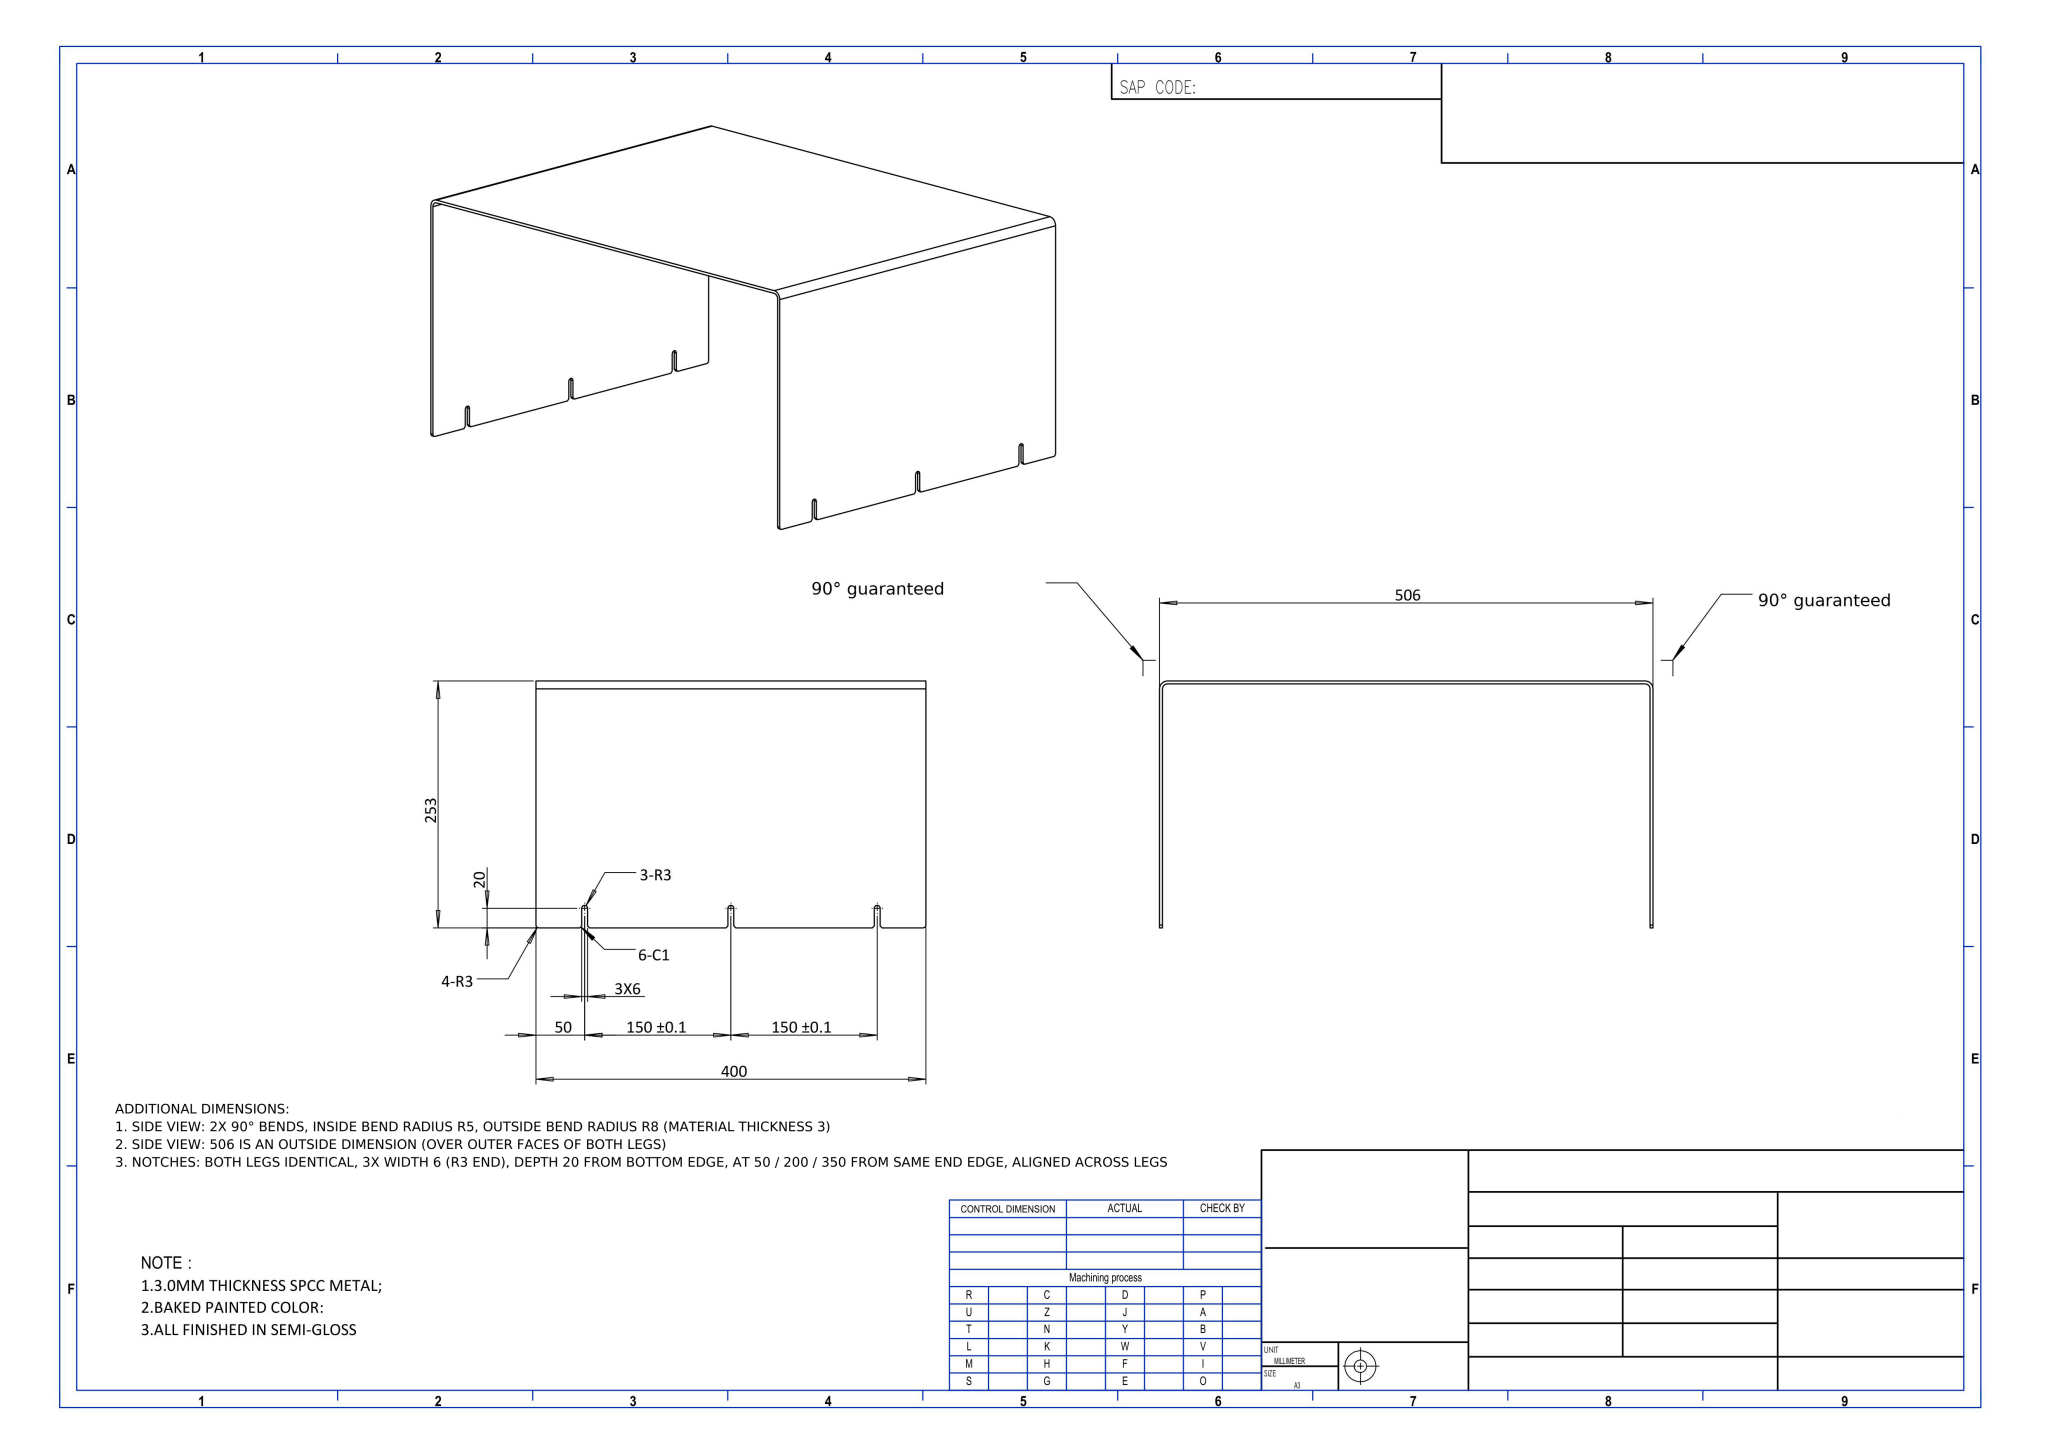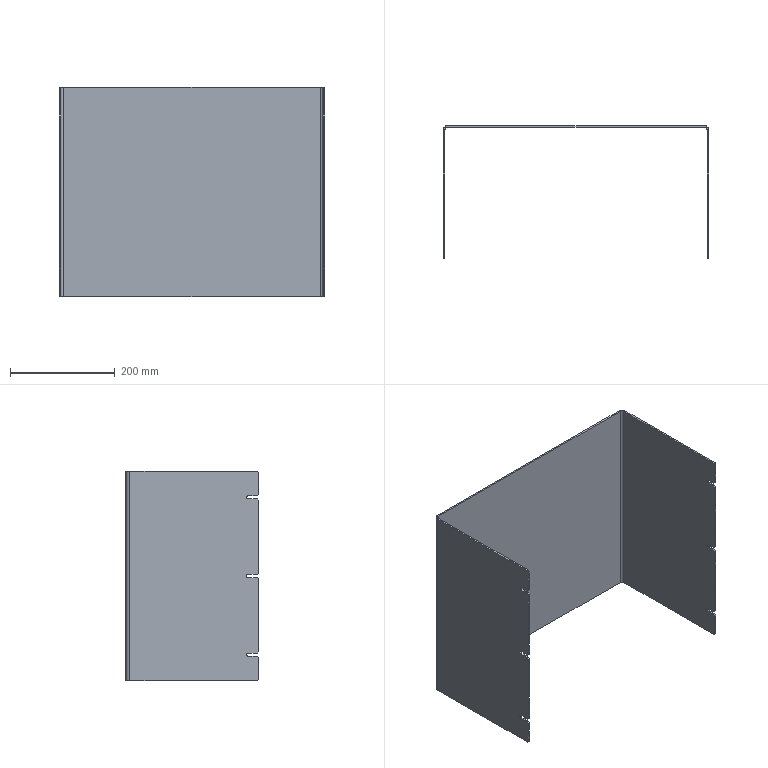Part | NX | mm | 1 solid | 54 faces | box 506 x 253 x 400 mm | volume 1197995 mm3 | plane 40 | cylinder 14 | commonest cylinder face diameters 6 x10 16 x2 10 x2